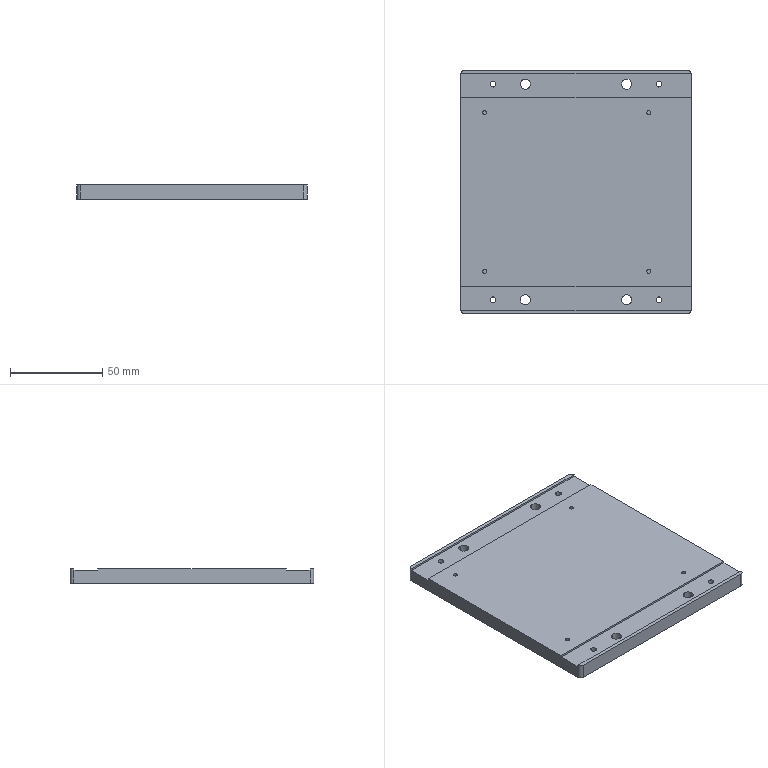CAM job | Mastercam | mm | 9 operations | part box 125 x 132 x 8
1. Facing | 20 - 63 平铣刀
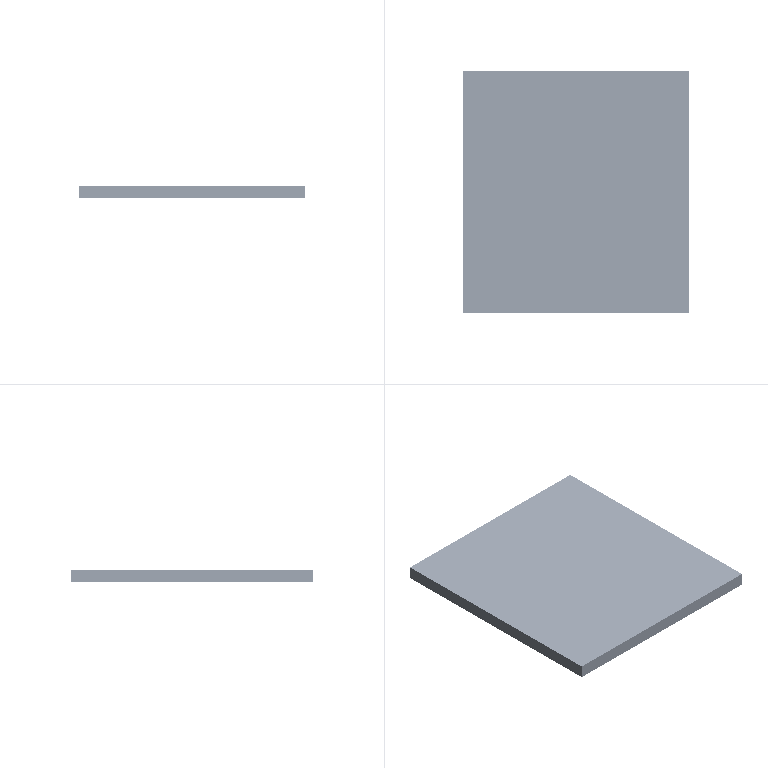2. 2D High Speed (2D Dynamic Mill) | 10 - 10 平铣刀
3. Contour (2D) | 10 - 10 平铣刀
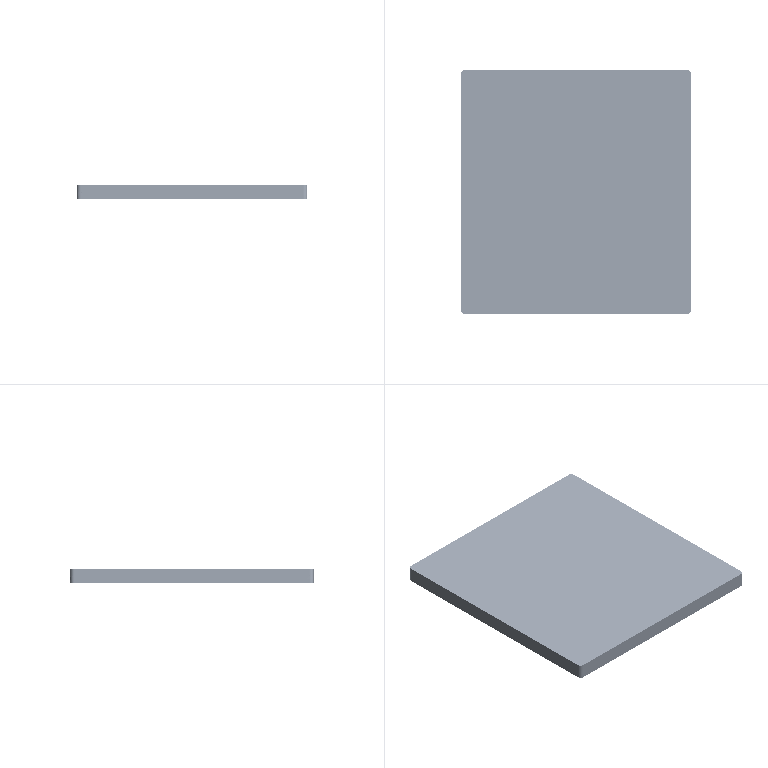4. Contour (2D chamfer) | 7 - 4 倒角刀
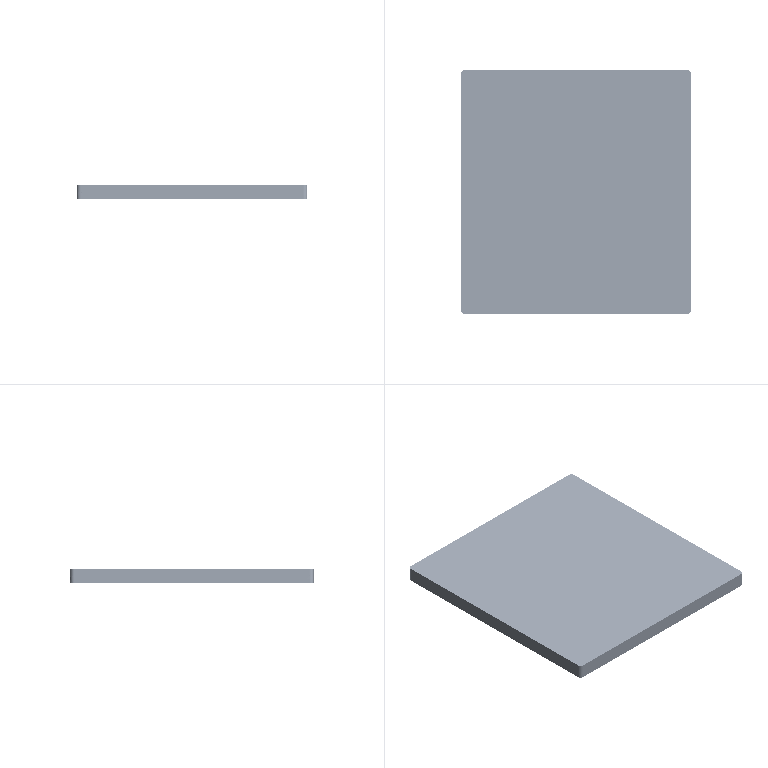5. Facing | 20 - 63 平铣刀
6. Contour (Ramp) | 10 - 10 平铣刀
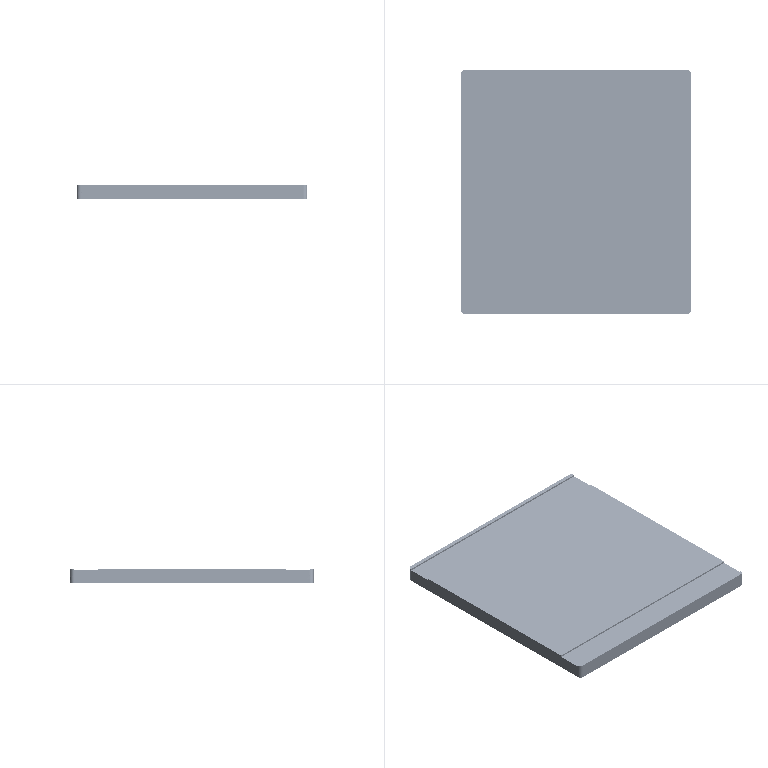7. Contour (2D) | 10 - 10 平铣刀
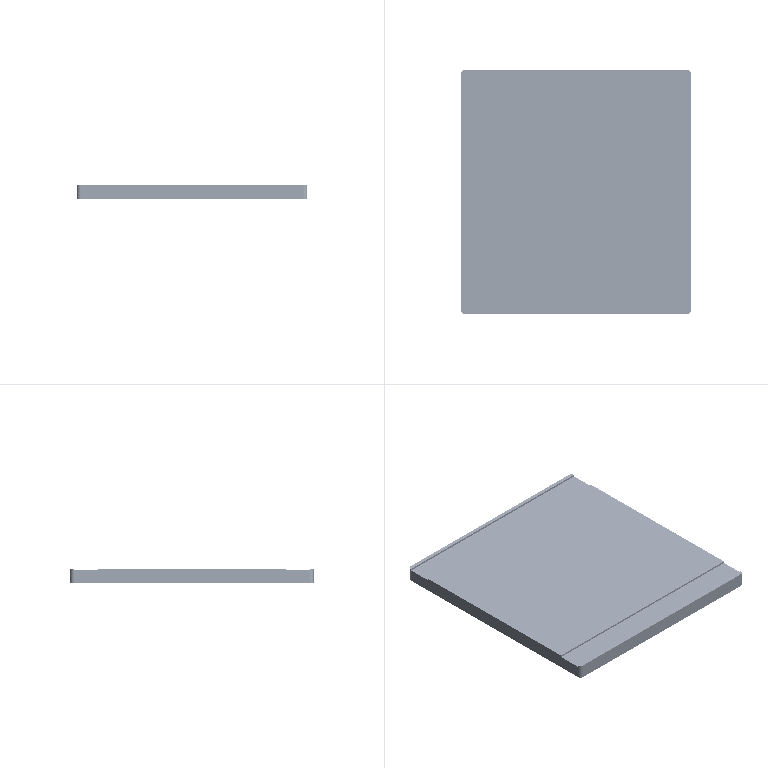8. Drill/Counterbore | 7 - 4 倒角刀
9. Contour (2D chamfer) | 7 - 4 倒角刀